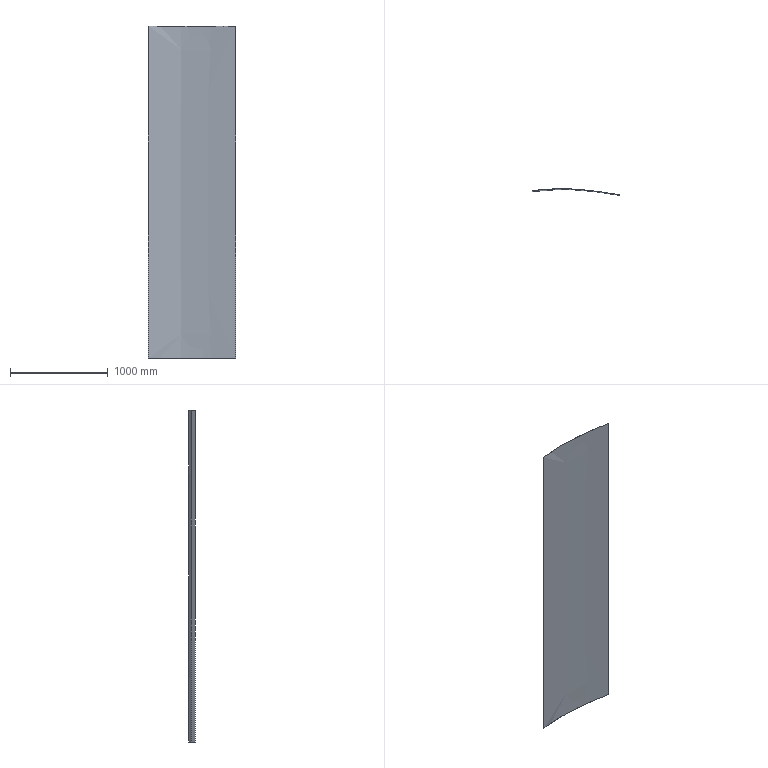Component | NX | SKIN_0_5_UPPER | 1 solid | 6 faces | box 890.47 x 63.54 x 3390 mm | volume 1517863 mm3 | plane 4 | other 2
STEP:
#1=CARTESIAN_POINT('',(0.,0.,0.));
#2=DIRECTION('',(0.,0.,1.));
#3=DIRECTION('',(1.,0.,0.));
#4=AXIS2_PLACEMENT_3D('',#1,#2,#3);
#5=CARTESIAN_POINT('',(5766.678,4293.299,-3390.));
#6=VERTEX_POINT('',#5);
#7=CARTESIAN_POINT('',(5766.787,4292.811,-3390.));
#8=VERTEX_POINT('',#7);
#9=CARTESIAN_POINT('',(5766.678,4293.299,-3390.));
#10=DIRECTION('',(0.2171,-0.9761,0.));
#11=VECTOR('',#10,1.);
#12=LINE('',#9,#11);
#13=CARTESIAN_POINT('',(5766.678,4293.299,0.));
#14=DIRECTION('',(0.9761,0.2171,0.));
#15=DIRECTION('',(-0.2171,0.9761,0.));
#16=AXIS2_PLACEMENT_3D('',#13,#14,#15);
#17=PLANE('',#16);
#18=CARTESIAN_POINT('',(0.,-3390.));
#19=DIRECTION('',(-1.,0.));
#20=VECTOR('',#19,1.);
#21=LINE('',#18,#20);
#22=(GEOMETRIC_REPRESENTATION_CONTEXT(2)PARAMETRIC_REPRESENTATION_CONTEXT()REPRESENTATION_CONTEXT('',''));
#23=DEFINITIONAL_REPRESENTATION('',(#21),#22);
#24=PCURVE('',#17,#23);
#25=CARTESIAN_POINT('',(6213.134,4311.301,-3390.));
#26=DIRECTION('',(0.,0.,1.));
#27=DIRECTION('',(1.,0.008727,0.));
#28=AXIS2_PLACEMENT_3D('',#25,#26,#27);
#29=PLANE('',#28);
#30=CARTESIAN_POINT('',(-446.596,-14.105));
#31=DIRECTION('',(0.2086,-0.978));
#32=VECTOR('',#31,1.);
#33=LINE('',#30,#32);
#34=(GEOMETRIC_REPRESENTATION_CONTEXT(2)PARAMETRIC_REPRESENTATION_CONTEXT()REPRESENTATION_CONTEXT('',''));
#35=DEFINITIONAL_REPRESENTATION('',(#33),#34);
#36=PCURVE('',#29,#35);
#37=SURFACE_CURVE('',#12,(#24,#36),.PCURVE_S1.);
#38=EDGE_CURVE('',#6,#8,#37,.T.);
#39=ORIENTED_EDGE('',*,*,#38,.T.);
#40=CARTESIAN_POINT('',(5766.787,4292.811,0.));
#41=VERTEX_POINT('',#40);
#42=CARTESIAN_POINT('',(5766.787,4292.811,0.));
#43=DIRECTION('',(0.,0.,-1.));
#44=VECTOR('',#43,1.);
#45=LINE('',#42,#44);
#46=CARTESIAN_POINT('',(-0.5,0.));
#47=DIRECTION('',(0.,-1.));
#48=VECTOR('',#47,1.);
#49=LINE('',#46,#48);
#50=(GEOMETRIC_REPRESENTATION_CONTEXT(2)PARAMETRIC_REPRESENTATION_CONTEXT()REPRESENTATION_CONTEXT('',''));
#51=DEFINITIONAL_REPRESENTATION('',(#49),#50);
#52=PCURVE('',#17,#51);
#53=CARTESIAN_POINT('',(5766.787,4292.811,0.));
#54=CARTESIAN_POINT('',(5803.405,4300.955,0.));
#55=CARTESIAN_POINT('',(5840.426,4305.181,0.));
#56=CARTESIAN_POINT('',(5896.21,4309.297,0.));
#57=CARTESIAN_POINT('',(5914.846,4310.299,0.));
#58=CARTESIAN_POINT('',(5938.157,4311.471,0.));
#59=CARTESIAN_POINT('',(5942.82,4311.701,0.));
#60=CARTESIAN_POINT('',(5952.146,4312.161,0.));
#61=CARTESIAN_POINT('',(5966.136,4312.847,0.));
#62=CARTESIAN_POINT('',(5980.128,4313.499,0.));
#63=CARTESIAN_POINT('',(6026.767,4315.528,0.));
#64=CARTESIAN_POINT('',(6064.08,4316.678,0.));
#65=CARTESIAN_POINT('',(6110.687,4316.309,0.));
#66=CARTESIAN_POINT('',(6120.006,4316.142,0.));
#67=CARTESIAN_POINT('',(6138.641,4315.611,0.));
#68=CARTESIAN_POINT('',(6166.59,4314.532,0.));
#69=CARTESIAN_POINT('',(6213.143,4311.517,0.));
#70=CARTESIAN_POINT('',(6250.35,4308.241,0.));
#71=CARTESIAN_POINT('',(6278.24,4305.622,0.));
#72=CARTESIAN_POINT('',(6287.534,4304.724,0.));
#73=CARTESIAN_POINT('',(6306.115,4302.888,0.));
#74=CARTESIAN_POINT('',(6352.554,4298.193,0.));
#75=CARTESIAN_POINT('',(6398.908,4292.921,0.));
#76=CARTESIAN_POINT('',(6509.95,4278.825,0.));
#77=CARTESIAN_POINT('',(6583.701,4267.509,0.));
#78=CARTESIAN_POINT('',(6657.05,4253.392,0.));
#79=B_SPLINE_CURVE_WITH_KNOTS('',3,(#53,#54,#55,#56,#57,#58,#59,#60,#61,#62,#63,#64,#65,#66,#67,#68,#69,#70,#71,#72,#73,#74,#75,#76,#77,#78),.UNSPECIFIED.,.F.,.F.,(4,2,2,2,1,2,2,2,1,1,2,2,1,2,4),(0.,0.125,0.1875,0.2031,0.2188,0.25,0.375,0.4062,0.4375,0.5,0.5625,0.5938,0.625,0.75,1.),.UNSPECIFIED.);
#80=DIRECTION('',(0.,0.,-1.));
#81=VECTOR('',#80,1.);
#82=SURFACE_OF_LINEAR_EXTRUSION('',#79,#81);
#83=CARTESIAN_POINT('',(0.,0.));
#84=DIRECTION('',(-0.,1.));
#85=VECTOR('',#84,1.);
#86=LINE('',#83,#85);
#87=(GEOMETRIC_REPRESENTATION_CONTEXT(2)PARAMETRIC_REPRESENTATION_CONTEXT()REPRESENTATION_CONTEXT('',''));
#88=DEFINITIONAL_REPRESENTATION('',(#86),#87);
#89=PCURVE('',#82,#88);
#90=SURFACE_CURVE('',#45,(#52,#89),.PCURVE_S1.);
#91=EDGE_CURVE('',#41,#8,#90,.T.);
#92=ORIENTED_EDGE('',*,*,#91,.F.);
#93=CARTESIAN_POINT('',(5766.678,4293.299,0.));
#94=VERTEX_POINT('',#93);
#95=CARTESIAN_POINT('',(5766.678,4293.299,0.));
#96=DIRECTION('',(0.2171,-0.9761,0.));
#97=VECTOR('',#96,1.);
#98=LINE('',#95,#97);
#99=CARTESIAN_POINT('',(0.,0.));
#100=DIRECTION('',(-1.,0.));
#101=VECTOR('',#100,1.);
#102=LINE('',#99,#101);
#103=(GEOMETRIC_REPRESENTATION_CONTEXT(2)PARAMETRIC_REPRESENTATION_CONTEXT()REPRESENTATION_CONTEXT('',''));
#104=DEFINITIONAL_REPRESENTATION('',(#102),#103);
#105=PCURVE('',#17,#104);
#106=CARTESIAN_POINT('',(6213.134,4311.301,0.));
#107=DIRECTION('',(0.,0.,1.));
#108=DIRECTION('',(1.,0.008727,0.));
#109=AXIS2_PLACEMENT_3D('',#106,#107,#108);
#110=PLANE('',#109);
#111=CARTESIAN_POINT('',(-446.596,-14.105));
#112=DIRECTION('',(0.2086,-0.978));
#113=VECTOR('',#112,1.);
#114=LINE('',#111,#113);
#115=(GEOMETRIC_REPRESENTATION_CONTEXT(2)PARAMETRIC_REPRESENTATION_CONTEXT()REPRESENTATION_CONTEXT('',''));
#116=DEFINITIONAL_REPRESENTATION('',(#114),#115);
#117=PCURVE('',#110,#116);
#118=SURFACE_CURVE('',#98,(#105,#117),.PCURVE_S1.);
#119=EDGE_CURVE('',#94,#41,#118,.T.);
#120=ORIENTED_EDGE('',*,*,#119,.F.);
#121=CARTESIAN_POINT('',(5766.678,4293.299,0.));
#122=DIRECTION('',(0.,0.,-1.));
#123=VECTOR('',#122,1.);
#124=LINE('',#121,#123);
#125=CARTESIAN_POINT('',(0.,0.));
#126=DIRECTION('',(0.,-1.));
#127=VECTOR('',#126,1.);
#128=LINE('',#125,#127);
#129=(GEOMETRIC_REPRESENTATION_CONTEXT(2)PARAMETRIC_REPRESENTATION_CONTEXT()REPRESENTATION_CONTEXT('',''));
#130=DEFINITIONAL_REPRESENTATION('',(#128),#129);
#131=PCURVE('',#17,#130);
#132=CARTESIAN_POINT('',(6657.145,4253.882,0.));
#133=CARTESIAN_POINT('',(6533.16,4277.746,0.));
#134=CARTESIAN_POINT('',(6353.754,4300.487,0.));
#135=CARTESIAN_POINT('',(6114.639,4320.403,0.));
#136=CARTESIAN_POINT('',(5942.157,4312.33,0.));
#137=CARTESIAN_POINT('',(5824.608,4306.183,0.));
#138=CARTESIAN_POINT('',(5766.678,4293.299,0.));
#139=B_SPLINE_CURVE_WITH_KNOTS('',3,(#132,#133,#134,#135,#136,#137,#138),.UNSPECIFIED.,.F.,.F.,(4,1,1,1,4),(0.,0.4225,0.6058,0.8024,1.),.UNSPECIFIED.);
#140=DIRECTION('',(0.,0.,-1.));
#141=VECTOR('',#140,1.);
#142=SURFACE_OF_LINEAR_EXTRUSION('',#139,#141);
#143=CARTESIAN_POINT('',(1.,0.));
#144=DIRECTION('',(0.,1.));
#145=VECTOR('',#144,1.);
#146=LINE('',#143,#145);
#147=(GEOMETRIC_REPRESENTATION_CONTEXT(2)PARAMETRIC_REPRESENTATION_CONTEXT()REPRESENTATION_CONTEXT('',''));
#148=DEFINITIONAL_REPRESENTATION('',(#146),#147);
#149=PCURVE('',#142,#148);
#150=SURFACE_CURVE('',#124,(#131,#149),.PCURVE_S1.);
#151=EDGE_CURVE('',#94,#6,#150,.T.);
#152=ORIENTED_EDGE('',*,*,#151,.T.);
#153=EDGE_LOOP('',(#39,#92,#120,#152));
#154=FACE_BOUND('',#153,.T.);
#155=ADVANCED_FACE('',(#154),#17,.F.);
#156=ORIENTED_EDGE('',*,*,#91,.F.);
#157=CARTESIAN_POINT('',(6657.05,4253.392,0.));
#158=VERTEX_POINT('',#157);
#159=CARTESIAN_POINT('',(5766.787,4292.811,0.));
#160=CARTESIAN_POINT('',(5803.405,4300.955,0.));
#161=CARTESIAN_POINT('',(5840.426,4305.181,0.));
#162=CARTESIAN_POINT('',(5896.21,4309.297,0.));
#163=CARTESIAN_POINT('',(5914.846,4310.299,0.));
#164=CARTESIAN_POINT('',(5938.157,4311.471,0.));
#165=CARTESIAN_POINT('',(5942.82,4311.701,0.));
#166=CARTESIAN_POINT('',(5952.146,4312.161,0.));
#167=CARTESIAN_POINT('',(5966.136,4312.847,0.));
#168=CARTESIAN_POINT('',(5980.128,4313.499,0.));
#169=CARTESIAN_POINT('',(6026.767,4315.528,0.));
#170=CARTESIAN_POINT('',(6064.08,4316.678,0.));
#171=CARTESIAN_POINT('',(6110.687,4316.309,0.));
#172=CARTESIAN_POINT('',(6120.006,4316.142,0.));
#173=CARTESIAN_POINT('',(6138.641,4315.611,0.));
#174=CARTESIAN_POINT('',(6166.59,4314.532,0.));
#175=CARTESIAN_POINT('',(6213.143,4311.517,0.));
#176=CARTESIAN_POINT('',(6250.35,4308.241,0.));
#177=CARTESIAN_POINT('',(6278.24,4305.622,0.));
#178=CARTESIAN_POINT('',(6287.534,4304.724,0.));
#179=CARTESIAN_POINT('',(6306.115,4302.888,0.));
#180=CARTESIAN_POINT('',(6352.554,4298.193,0.));
#181=CARTESIAN_POINT('',(6398.908,4292.921,0.));
#182=CARTESIAN_POINT('',(6509.95,4278.825,0.));
#183=CARTESIAN_POINT('',(6583.701,4267.509,0.));
#184=CARTESIAN_POINT('',(6657.05,4253.392,0.));
#185=B_SPLINE_CURVE_WITH_KNOTS('',3,(#159,#160,#161,#162,#163,#164,#165,#166,#167,#168,#169,#170,#171,#172,#173,#174,#175,#176,#177,#178,#179,#180,#181,#182,#183,#184),.UNSPECIFIED.,.F.,.F.,(4,2,2,2,1,2,2,2,1,1,2,2,1,2,4),(0.,0.125,0.1875,0.2031,0.2188,0.25,0.375,0.4062,0.4375,0.5,0.5625,0.5938,0.625,0.75,1.),.UNSPECIFIED.);
#186=CARTESIAN_POINT('',(0.,0.));
#187=DIRECTION('',(1.,0.));
#188=VECTOR('',#187,1.);
#189=LINE('',#186,#188);
#190=(GEOMETRIC_REPRESENTATION_CONTEXT(2)PARAMETRIC_REPRESENTATION_CONTEXT()REPRESENTATION_CONTEXT('',''));
#191=DEFINITIONAL_REPRESENTATION('',(#189),#190);
#192=PCURVE('',#82,#191);
#193=CARTESIAN_POINT('',(-446.492,-14.594));
#194=CARTESIAN_POINT('',(-409.803,-6.77));
#195=CARTESIAN_POINT('',(-372.747,-2.868));
#196=CARTESIAN_POINT('',(-316.929,0.7623));
#197=CARTESIAN_POINT('',(-298.285,1.602));
#198=CARTESIAN_POINT('',(-274.965,2.57));
#199=CARTESIAN_POINT('',(-270.3,2.76));
#200=CARTESIAN_POINT('',(-260.97,3.138));
#201=CARTESIAN_POINT('',(-246.975,3.701));
#202=CARTESIAN_POINT('',(-232.978,4.232));
#203=CARTESIAN_POINT('',(-186.323,5.854));
#204=CARTESIAN_POINT('',(-149.001,6.678));
#205=CARTESIAN_POINT('',(-102.4,5.902));
#206=CARTESIAN_POINT('',(-93.082,5.654));
#207=CARTESIAN_POINT('',(-74.452,4.961));
#208=CARTESIAN_POINT('',(-46.514,3.637));
#209=CARTESIAN_POINT('',(0.01076,0.2159));
#210=CARTESIAN_POINT('',(37.188,-3.385));
#211=CARTESIAN_POINT('',(65.054,-6.247));
#212=CARTESIAN_POINT('',(74.339,-7.226));
#213=CARTESIAN_POINT('',(92.904,-9.223));
#214=CARTESIAN_POINT('',(139.3,-14.323));
#215=CARTESIAN_POINT('',(185.606,-20.001));
#216=CARTESIAN_POINT('',(296.522,-35.064));
#217=CARTESIAN_POINT('',(370.171,-47.024));
#218=CARTESIAN_POINT('',(443.394,-61.781));
#219=B_SPLINE_CURVE_WITH_KNOTS('',3,(#193,#194,#195,#196,#197,#198,#199,#200,#201,#202,#203,#204,#205,#206,#207,#208,#209,#210,#211,#212,#213,#214,#215,#216,#217,#218),.UNSPECIFIED.,.F.,.F.,(4,2,2,2,1,2,2,2,1,1,2,2,1,2,4),(0.,0.125,0.1875,0.2031,0.2188,0.25,0.375,0.4062,0.4375,0.5,0.5625,0.5938,0.625,0.75,1.),.UNSPECIFIED.);
#220=(GEOMETRIC_REPRESENTATION_CONTEXT(2)PARAMETRIC_REPRESENTATION_CONTEXT()REPRESENTATION_CONTEXT('',''));
#221=DEFINITIONAL_REPRESENTATION('',(#219),#220);
#222=PCURVE('',#110,#221);
#223=SURFACE_CURVE('',#185,(#192,#222),.PCURVE_S1.);
#224=EDGE_CURVE('',#41,#158,#223,.T.);
#225=ORIENTED_EDGE('',*,*,#224,.T.);
#226=CARTESIAN_POINT('',(6657.05,4253.392,-3390.));
#227=VERTEX_POINT('',#226);
#228=CARTESIAN_POINT('',(6657.05,4253.392,0.));
#229=DIRECTION('',(0.,0.,-1.));
#230=VECTOR('',#229,1.);
#231=LINE('',#228,#230);
#232=CARTESIAN_POINT('',(1.,0.));
#233=DIRECTION('',(0.,1.));
#234=VECTOR('',#233,1.);
#235=LINE('',#232,#234);
#236=(GEOMETRIC_REPRESENTATION_CONTEXT(2)PARAMETRIC_REPRESENTATION_CONTEXT()REPRESENTATION_CONTEXT('',''));
#237=DEFINITIONAL_REPRESENTATION('',(#235),#236);
#238=PCURVE('',#82,#237);
#239=CARTESIAN_POINT('',(6657.05,4253.392,0.));
#240=DIRECTION('',(-0.982,0.189,0.));
#241=DIRECTION('',(-0.189,-0.982,0.));
#242=AXIS2_PLACEMENT_3D('',#239,#240,#241);
#243=PLANE('',#242);
#244=CARTESIAN_POINT('',(0.,0.));
#245=DIRECTION('',(0.,-1.));
#246=VECTOR('',#245,1.);
#247=LINE('',#244,#246);
#248=(GEOMETRIC_REPRESENTATION_CONTEXT(2)PARAMETRIC_REPRESENTATION_CONTEXT()REPRESENTATION_CONTEXT('',''));
#249=DEFINITIONAL_REPRESENTATION('',(#247),#248);
#250=PCURVE('',#243,#249);
#251=SURFACE_CURVE('',#231,(#238,#250),.PCURVE_S1.);
#252=EDGE_CURVE('',#158,#227,#251,.T.);
#253=ORIENTED_EDGE('',*,*,#252,.T.);
#254=CARTESIAN_POINT('',(5766.787,4292.811,-3390.));
#255=CARTESIAN_POINT('',(5803.405,4300.955,-3390.));
#256=CARTESIAN_POINT('',(5840.426,4305.181,-3390.));
#257=CARTESIAN_POINT('',(5896.21,4309.297,-3390.));
#258=CARTESIAN_POINT('',(5914.846,4310.299,-3390.));
#259=CARTESIAN_POINT('',(5938.157,4311.471,-3390.));
#260=CARTESIAN_POINT('',(5942.82,4311.701,-3390.));
#261=CARTESIAN_POINT('',(5952.146,4312.161,-3390.));
#262=CARTESIAN_POINT('',(5966.136,4312.847,-3390.));
#263=CARTESIAN_POINT('',(5980.128,4313.499,-3390.));
#264=CARTESIAN_POINT('',(6026.767,4315.528,-3390.));
#265=CARTESIAN_POINT('',(6064.08,4316.678,-3390.));
#266=CARTESIAN_POINT('',(6110.687,4316.309,-3390.));
#267=CARTESIAN_POINT('',(6120.006,4316.142,-3390.));
#268=CARTESIAN_POINT('',(6138.641,4315.611,-3390.));
#269=CARTESIAN_POINT('',(6166.59,4314.532,-3390.));
#270=CARTESIAN_POINT('',(6213.143,4311.517,-3390.));
#271=CARTESIAN_POINT('',(6250.35,4308.241,-3390.));
#272=CARTESIAN_POINT('',(6278.24,4305.622,-3390.));
#273=CARTESIAN_POINT('',(6287.534,4304.724,-3390.));
#274=CARTESIAN_POINT('',(6306.115,4302.888,-3390.));
#275=CARTESIAN_POINT('',(6352.554,4298.193,-3390.));
#276=CARTESIAN_POINT('',(6398.908,4292.921,-3390.));
#277=CARTESIAN_POINT('',(6509.95,4278.825,-3390.));
#278=CARTESIAN_POINT('',(6583.701,4267.509,-3390.));
#279=CARTESIAN_POINT('',(6657.05,4253.392,-3390.));
#280=B_SPLINE_CURVE_WITH_KNOTS('',3,(#254,#255,#256,#257,#258,#259,#260,#261,#262,#263,#264,#265,#266,#267,#268,#269,#270,#271,#272,#273,#274,#275,#276,#277,#278,#279),.UNSPECIFIED.,.F.,.F.,(4,2,2,2,1,2,2,2,1,1,2,2,1,2,4),(0.,0.125,0.1875,0.2031,0.2188,0.25,0.375,0.4062,0.4375,0.5,0.5625,0.5938,0.625,0.75,1.),.UNSPECIFIED.);
#281=CARTESIAN_POINT('',(-0.,3390.));
#282=DIRECTION('',(1.,0.));
#283=VECTOR('',#282,1.);
#284=LINE('',#281,#283);
#285=(GEOMETRIC_REPRESENTATION_CONTEXT(2)PARAMETRIC_REPRESENTATION_CONTEXT()REPRESENTATION_CONTEXT('',''));
#286=DEFINITIONAL_REPRESENTATION('',(#284),#285);
#287=PCURVE('',#82,#286);
#288=CARTESIAN_POINT('',(-446.492,-14.594));
#289=CARTESIAN_POINT('',(-409.803,-6.77));
#290=CARTESIAN_POINT('',(-372.747,-2.868));
#291=CARTESIAN_POINT('',(-316.929,0.7623));
#292=CARTESIAN_POINT('',(-298.285,1.602));
#293=CARTESIAN_POINT('',(-274.965,2.57));
#294=CARTESIAN_POINT('',(-270.3,2.76));
#295=CARTESIAN_POINT('',(-260.97,3.138));
#296=CARTESIAN_POINT('',(-246.975,3.701));
#297=CARTESIAN_POINT('',(-232.978,4.232));
#298=CARTESIAN_POINT('',(-186.323,5.854));
#299=CARTESIAN_POINT('',(-149.001,6.678));
#300=CARTESIAN_POINT('',(-102.4,5.902));
#301=CARTESIAN_POINT('',(-93.082,5.654));
#302=CARTESIAN_POINT('',(-74.452,4.961));
#303=CARTESIAN_POINT('',(-46.514,3.637));
#304=CARTESIAN_POINT('',(0.01076,0.2159));
#305=CARTESIAN_POINT('',(37.188,-3.385));
#306=CARTESIAN_POINT('',(65.054,-6.247));
#307=CARTESIAN_POINT('',(74.339,-7.226));
#308=CARTESIAN_POINT('',(92.904,-9.223));
#309=CARTESIAN_POINT('',(139.3,-14.323));
#310=CARTESIAN_POINT('',(185.606,-20.001));
#311=CARTESIAN_POINT('',(296.522,-35.064));
#312=CARTESIAN_POINT('',(370.171,-47.024));
#313=CARTESIAN_POINT('',(443.394,-61.781));
#314=B_SPLINE_CURVE_WITH_KNOTS('',3,(#288,#289,#290,#291,#292,#293,#294,#295,#296,#297,#298,#299,#300,#301,#302,#303,#304,#305,#306,#307,#308,#309,#310,#311,#312,#313),.UNSPECIFIED.,.F.,.F.,(4,2,2,2,1,2,2,2,1,1,2,2,1,2,4),(0.,0.125,0.1875,0.2031,0.2188,0.25,0.375,0.4062,0.4375,0.5,0.5625,0.5938,0.625,0.75,1.),.UNSPECIFIED.);
#315=(GEOMETRIC_REPRESENTATION_CONTEXT(2)PARAMETRIC_REPRESENTATION_CONTEXT()REPRESENTATION_CONTEXT('',''));
#316=DEFINITIONAL_REPRESENTATION('',(#314),#315);
#317=PCURVE('',#29,#316);
#318=SURFACE_CURVE('',#280,(#287,#317),.PCURVE_S1.);
#319=EDGE_CURVE('',#8,#227,#318,.T.);
#320=ORIENTED_EDGE('',*,*,#319,.F.);
#321=EDGE_LOOP('',(#156,#225,#253,#320));
#322=FACE_BOUND('',#321,.F.);
#323=ADVANCED_FACE('',(#322),#82,.F.);
#324=CARTESIAN_POINT('',(6657.145,4253.882,-3390.));
#325=VERTEX_POINT('',#324);
#326=CARTESIAN_POINT('',(6657.05,4253.392,-3390.));
#327=DIRECTION('',(0.189,0.982,0.));
#328=VECTOR('',#327,1.);
#329=LINE('',#326,#328);
#330=CARTESIAN_POINT('',(0.,-3390.));
#331=DIRECTION('',(-1.,0.));
#332=VECTOR('',#331,1.);
#333=LINE('',#330,#332);
#334=(GEOMETRIC_REPRESENTATION_CONTEXT(2)PARAMETRIC_REPRESENTATION_CONTEXT()REPRESENTATION_CONTEXT('',''));
#335=DEFINITIONAL_REPRESENTATION('',(#333),#334);
#336=PCURVE('',#243,#335);
#337=CARTESIAN_POINT('',(443.394,-61.781));
#338=DIRECTION('',(0.1976,0.9803));
#339=VECTOR('',#338,1.);
#340=LINE('',#337,#339);
#341=(GEOMETRIC_REPRESENTATION_CONTEXT(2)PARAMETRIC_REPRESENTATION_CONTEXT()REPRESENTATION_CONTEXT('',''));
#342=DEFINITIONAL_REPRESENTATION('',(#340),#341);
#343=PCURVE('',#29,#342);
#344=SURFACE_CURVE('',#329,(#336,#343),.PCURVE_S1.);
#345=EDGE_CURVE('',#227,#325,#344,.T.);
#346=ORIENTED_EDGE('',*,*,#345,.T.);
#347=CARTESIAN_POINT('',(6657.145,4253.882,0.));
#348=VERTEX_POINT('',#347);
#349=CARTESIAN_POINT('',(6657.145,4253.882,0.));
#350=DIRECTION('',(0.,0.,-1.));
#351=VECTOR('',#350,1.);
#352=LINE('',#349,#351);
#353=CARTESIAN_POINT('',(-0.5,0.));
#354=DIRECTION('',(0.,-1.));
#355=VECTOR('',#354,1.);
#356=LINE('',#353,#355);
#357=(GEOMETRIC_REPRESENTATION_CONTEXT(2)PARAMETRIC_REPRESENTATION_CONTEXT()REPRESENTATION_CONTEXT('',''));
#358=DEFINITIONAL_REPRESENTATION('',(#356),#357);
#359=PCURVE('',#243,#358);
#360=CARTESIAN_POINT('',(-0.,0.));
#361=DIRECTION('',(0.,1.));
#362=VECTOR('',#361,1.);
#363=LINE('',#360,#362);
#364=(GEOMETRIC_REPRESENTATION_CONTEXT(2)PARAMETRIC_REPRESENTATION_CONTEXT()REPRESENTATION_CONTEXT('',''));
#365=DEFINITIONAL_REPRESENTATION('',(#363),#364);
#366=PCURVE('',#142,#365);
#367=SURFACE_CURVE('',#352,(#359,#366),.PCURVE_S1.);
#368=EDGE_CURVE('',#348,#325,#367,.T.);
#369=ORIENTED_EDGE('',*,*,#368,.F.);
#370=CARTESIAN_POINT('',(6657.05,4253.392,0.));
#371=DIRECTION('',(0.189,0.982,0.));
#372=VECTOR('',#371,1.);
#373=LINE('',#370,#372);
#374=CARTESIAN_POINT('',(0.,0.));
#375=DIRECTION('',(-1.,0.));
#376=VECTOR('',#375,1.);
#377=LINE('',#374,#376);
#378=(GEOMETRIC_REPRESENTATION_CONTEXT(2)PARAMETRIC_REPRESENTATION_CONTEXT()REPRESENTATION_CONTEXT('',''));
#379=DEFINITIONAL_REPRESENTATION('',(#377),#378);
#380=PCURVE('',#243,#379);
#381=CARTESIAN_POINT('',(443.394,-61.781));
#382=DIRECTION('',(0.1976,0.9803));
#383=VECTOR('',#382,1.);
#384=LINE('',#381,#383);
#385=(GEOMETRIC_REPRESENTATION_CONTEXT(2)PARAMETRIC_REPRESENTATION_CONTEXT()REPRESENTATION_CONTEXT('',''));
#386=DEFINITIONAL_REPRESENTATION('',(#384),#385);
#387=PCURVE('',#110,#386);
#388=SURFACE_CURVE('',#373,(#380,#387),.PCURVE_S1.);
#389=EDGE_CURVE('',#158,#348,#388,.T.);
#390=ORIENTED_EDGE('',*,*,#389,.F.);
#391=ORIENTED_EDGE('',*,*,#252,.T.);
#392=EDGE_LOOP('',(#346,#369,#390,#391));
#393=FACE_BOUND('',#392,.T.);
#394=ADVANCED_FACE('',(#393),#243,.F.);
#395=ORIENTED_EDGE('',*,*,#368,.F.);
#396=CARTESIAN_POINT('',(6657.145,4253.882,0.));
#397=CARTESIAN_POINT('',(6533.16,4277.746,0.));
#398=CARTESIAN_POINT('',(6353.754,4300.487,0.));
#399=CARTESIAN_POINT('',(6114.639,4320.403,0.));
#400=CARTESIAN_POINT('',(5942.157,4312.33,0.));
#401=CARTESIAN_POINT('',(5824.608,4306.183,0.));
#402=CARTESIAN_POINT('',(5766.678,4293.299,0.));
#403=B_SPLINE_CURVE_WITH_KNOTS('',3,(#396,#397,#398,#399,#400,#401,#402),.UNSPECIFIED.,.F.,.F.,(4,1,1,1,4),(0.,0.4225,0.6058,0.8024,1.),.UNSPECIFIED.);
#404=CARTESIAN_POINT('',(-0.,0.));
#405=DIRECTION('',(1.,0.));
#406=VECTOR('',#405,1.);
#407=LINE('',#404,#406);
#408=(GEOMETRIC_REPRESENTATION_CONTEXT(2)PARAMETRIC_REPRESENTATION_CONTEXT()REPRESENTATION_CONTEXT('',''));
#409=DEFINITIONAL_REPRESENTATION('',(#407),#408);
#410=PCURVE('',#142,#409);
#411=CARTESIAN_POINT('',(443.493,-61.291));
#412=CARTESIAN_POINT('',(319.721,-36.346));
#413=CARTESIAN_POINT('',(140.521,-12.04));
#414=CARTESIAN_POINT('',(-98.411,9.961));
#415=CARTESIAN_POINT('',(-270.958,3.394));
#416=CARTESIAN_POINT('',(-388.556,-1.727));
#417=CARTESIAN_POINT('',(-446.596,-14.105));
#418=B_SPLINE_CURVE_WITH_KNOTS('',3,(#411,#412,#413,#414,#415,#416,#417),.UNSPECIFIED.,.F.,.F.,(4,1,1,1,4),(0.,0.4225,0.6058,0.8024,1.),.UNSPECIFIED.);
#419=(GEOMETRIC_REPRESENTATION_CONTEXT(2)PARAMETRIC_REPRESENTATION_CONTEXT()REPRESENTATION_CONTEXT('',''));
#420=DEFINITIONAL_REPRESENTATION('',(#418),#419);
#421=PCURVE('',#110,#420);
#422=SURFACE_CURVE('',#403,(#410,#421),.PCURVE_S1.);
#423=EDGE_CURVE('',#348,#94,#422,.T.);
#424=ORIENTED_EDGE('',*,*,#423,.T.);
#425=ORIENTED_EDGE('',*,*,#151,.T.);
#426=CARTESIAN_POINT('',(6657.145,4253.882,-3390.));
#427=CARTESIAN_POINT('',(6533.16,4277.746,-3390.));
#428=CARTESIAN_POINT('',(6353.754,4300.487,-3390.));
#429=CARTESIAN_POINT('',(6114.639,4320.403,-3390.));
#430=CARTESIAN_POINT('',(5942.157,4312.33,-3390.));
#431=CARTESIAN_POINT('',(5824.608,4306.183,-3390.));
#432=CARTESIAN_POINT('',(5766.678,4293.299,-3390.));
#433=B_SPLINE_CURVE_WITH_KNOTS('',3,(#426,#427,#428,#429,#430,#431,#432),.UNSPECIFIED.,.F.,.F.,(4,1,1,1,4),(0.,0.4225,0.6058,0.8024,1.),.UNSPECIFIED.);
#434=CARTESIAN_POINT('',(0.,3390.));
#435=DIRECTION('',(1.,0.));
#436=VECTOR('',#435,1.);
#437=LINE('',#434,#436);
#438=(GEOMETRIC_REPRESENTATION_CONTEXT(2)PARAMETRIC_REPRESENTATION_CONTEXT()REPRESENTATION_CONTEXT('',''));
#439=DEFINITIONAL_REPRESENTATION('',(#437),#438);
#440=PCURVE('',#142,#439);
#441=CARTESIAN_POINT('',(443.493,-61.291));
#442=CARTESIAN_POINT('',(319.721,-36.346));
#443=CARTESIAN_POINT('',(140.521,-12.04));
#444=CARTESIAN_POINT('',(-98.411,9.961));
#445=CARTESIAN_POINT('',(-270.958,3.394));
#446=CARTESIAN_POINT('',(-388.556,-1.727));
#447=CARTESIAN_POINT('',(-446.596,-14.105));
#448=B_SPLINE_CURVE_WITH_KNOTS('',3,(#441,#442,#443,#444,#445,#446,#447),.UNSPECIFIED.,.F.,.F.,(4,1,1,1,4),(0.,0.4225,0.6058,0.8024,1.),.UNSPECIFIED.);
#449=(GEOMETRIC_REPRESENTATION_CONTEXT(2)PARAMETRIC_REPRESENTATION_CONTEXT()REPRESENTATION_CONTEXT('',''));
#450=DEFINITIONAL_REPRESENTATION('',(#448),#449);
#451=PCURVE('',#29,#450);
#452=SURFACE_CURVE('',#433,(#440,#451),.PCURVE_S1.);
#453=EDGE_CURVE('',#325,#6,#452,.T.);
#454=ORIENTED_EDGE('',*,*,#453,.F.);
#455=EDGE_LOOP('',(#395,#424,#425,#454));
#456=FACE_BOUND('',#455,.F.);
#457=ADVANCED_FACE('',(#456),#142,.F.);
#458=ORIENTED_EDGE('',*,*,#119,.T.);
#459=ORIENTED_EDGE('',*,*,#224,.T.);
#460=ORIENTED_EDGE('',*,*,#389,.T.);
#461=ORIENTED_EDGE('',*,*,#423,.T.);
#462=EDGE_LOOP('',(#458,#459,#460,#461));
#463=FACE_BOUND('',#462,.T.);
#464=ADVANCED_FACE('',(#463),#110,.T.);
#465=ORIENTED_EDGE('',*,*,#38,.F.);
#466=ORIENTED_EDGE('',*,*,#453,.F.);
#467=ORIENTED_EDGE('',*,*,#345,.F.);
#468=ORIENTED_EDGE('',*,*,#319,.F.);
#469=EDGE_LOOP('',(#465,#466,#467,#468));
#470=FACE_BOUND('',#469,.T.);
#471=ADVANCED_FACE('',(#470),#29,.F.);
#472=CLOSED_SHELL('',(#155,#323,#394,#457,#464,#471));
#473=MANIFOLD_SOLID_BREP('',#472);
#474=(LENGTH_UNIT()NAMED_UNIT(*)SI_UNIT(.MILLI.,.METRE.));
#475=UNCERTAINTY_MEASURE_WITH_UNIT(LENGTH_MEASURE(0.0000001),#474,'','');
#476=(NAMED_UNIT(*)PLANE_ANGLE_UNIT()SI_UNIT($,.RADIAN.));
#477=(NAMED_UNIT(*)SI_UNIT($,.STERADIAN.)SOLID_ANGLE_UNIT());
#478=(GEOMETRIC_REPRESENTATION_CONTEXT(3)GLOBAL_UNCERTAINTY_ASSIGNED_CONTEXT((#475))GLOBAL_UNIT_ASSIGNED_CONTEXT((#474,#476,#477))REPRESENTATION_CONTEXT('',''));
#479=ADVANCED_BREP_SHAPE_REPRESENTATION('',(#4,#473),#478);